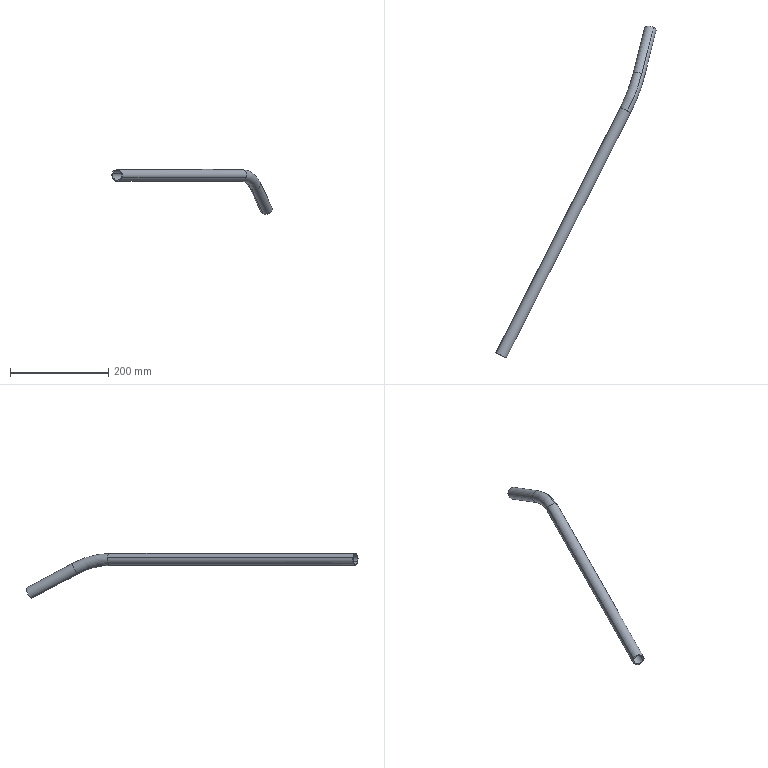Component | SolidWorks | ScribingMechanismAssembly-1_ScribingPlateMovableTube-1 | 1 solid | 14 faces | box 326.24 x 675.84 x 91.68 mm | volume 103418 mm3 | cylinder 8 | torus 4 | plane 2 | commonest cylinder face diameters 24 x4 20 x4
STEP:
#1=COLOUR_RGB('',0.7922,0.8196,0.9333);
#2=FILL_AREA_STYLE_COLOUR('',#1);
#3=FILL_AREA_STYLE('',(#2));
#4=SURFACE_STYLE_FILL_AREA(#3);
#5=SURFACE_SIDE_STYLE('',(#4));
#6=SURFACE_STYLE_USAGE(.BOTH.,#5);
#7=PRESENTATION_STYLE_ASSIGNMENT((#6));
#8=CARTESIAN_POINT('',(-5.227,-4.938,37.723));
#9=VERTEX_POINT('',#8);
#10=CARTESIAN_POINT('',(-5.042,-5.032,37.207));
#11=VERTEX_POINT('',#10);
#12=CARTESIAN_POINT('',(-5.365,-4.868,37.361));
#13=DIRECTION('',(0.4521,0.892,0.));
#14=DIRECTION('',(-0.8209,0.4161,0.3911));
#15=AXIS2_PLACEMENT_3D('',#12,#13,#14);
#16=CIRCLE('',#15,0.3937);
#17=EDGE_CURVE('',#9,#11,#16,.T.);
#18=ORIENTED_EDGE('',*,*,#17,.F.);
#19=CARTESIAN_POINT('',(-4.098,-1.979,36.947));
#20=VERTEX_POINT('',#19);
#21=CARTESIAN_POINT('',(-7.425,-3.824,31.926));
#22=DIRECTION('',(-0.8209,0.4161,0.3911));
#23=DIRECTION('',(-0.4521,-0.892,0.));
#24=AXIS2_PLACEMENT_3D('',#21,#22,#23);
#25=CIRCLE('',#24,6.299);
#26=EDGE_CURVE('',#9,#20,#25,.T.);
#27=ORIENTED_EDGE('',*,*,#26,.T.);
#28=CARTESIAN_POINT('',(-4.514,-2.21,36.319));
#29=VERTEX_POINT('',#28);
#30=CARTESIAN_POINT('',(-4.306,-2.095,36.633));
#31=DIRECTION('',(0.2171,0.8609,-0.4602));
#32=DIRECTION('',(-0.8209,0.4161,0.3911));
#33=AXIS2_PLACEMENT_3D('',#30,#31,#32);
#34=CIRCLE('',#33,0.3937);
#35=EDGE_CURVE('',#20,#29,#34,.T.);
#36=ORIENTED_EDGE('',*,*,#35,.T.);
#37=CARTESIAN_POINT('',(-5.502,-4.799,36.999));
#38=VERTEX_POINT('',#37);
#39=CARTESIAN_POINT('',(-7.425,-3.824,31.926));
#40=DIRECTION('',(-0.8209,0.4161,0.3911));
#41=DIRECTION('',(-0.4521,-0.892,0.));
#42=AXIS2_PLACEMENT_3D('',#39,#40,#41);
#43=CIRCLE('',#42,5.512);
#44=EDGE_CURVE('',#38,#29,#43,.T.);
#45=ORIENTED_EDGE('',*,*,#44,.F.);
#46=CARTESIAN_POINT('',(-5.365,-4.868,37.361));
#47=DIRECTION('',(0.4521,0.892,0.));
#48=DIRECTION('',(-0.8209,0.4161,0.3911));
#49=AXIS2_PLACEMENT_3D('',#46,#47,#48);
#50=CIRCLE('',#49,0.3937);
#51=EDGE_CURVE('',#11,#38,#50,.T.);
#52=ORIENTED_EDGE('',*,*,#51,.F.);
#53=EDGE_LOOP('',(#18,#27,#36,#45,#52));
#54=FACE_OUTER_BOUND('',#53,.T.);
#55=CARTESIAN_POINT('',(-7.425,-3.824,31.926));
#56=DIRECTION('',(-0.8209,0.4161,0.3911));
#57=DIRECTION('',(0.3489,-0.1768,0.9203));
#58=AXIS2_PLACEMENT_3D('',#55,#56,#57);
#59=TOROIDAL_SURFACE('',#58,5.906,0.3937);
#60=ADVANCED_FACE('',(#54),#59,.F.);
#61=CARTESIAN_POINT('',(-5.753,-4.672,37.546));
#62=VERTEX_POINT('',#61);
#63=CARTESIAN_POINT('',(-5.2,-4.952,37.796));
#64=VERTEX_POINT('',#63);
#65=CARTESIAN_POINT('',(-5.365,-4.868,37.361));
#66=DIRECTION('',(0.4521,0.892,0.));
#67=DIRECTION('',(-0.8209,0.4161,0.3911));
#68=AXIS2_PLACEMENT_3D('',#65,#66,#67);
#69=CIRCLE('',#68,0.4724);
#70=EDGE_CURVE('',#62,#64,#69,.T.);
#71=ORIENTED_EDGE('',*,*,#70,.T.);
#72=CARTESIAN_POINT('',(-4.056,-1.956,37.009));
#73=VERTEX_POINT('',#72);
#74=CARTESIAN_POINT('',(-7.425,-3.824,31.926));
#75=DIRECTION('',(-0.8209,0.4161,0.3911));
#76=DIRECTION('',(-0.4521,-0.892,0.));
#77=AXIS2_PLACEMENT_3D('',#74,#75,#76);
#78=CIRCLE('',#77,6.378);
#79=EDGE_CURVE('',#64,#73,#78,.T.);
#80=ORIENTED_EDGE('',*,*,#79,.T.);
#81=CARTESIAN_POINT('',(-4.555,-2.233,36.256));
#82=VERTEX_POINT('',#81);
#83=CARTESIAN_POINT('',(-4.306,-2.095,36.633));
#84=DIRECTION('',(0.2171,0.8609,-0.4602));
#85=DIRECTION('',(-0.8209,0.4161,0.3911));
#86=AXIS2_PLACEMENT_3D('',#83,#84,#85);
#87=CIRCLE('',#86,0.4724);
#88=EDGE_CURVE('',#82,#73,#87,.T.);
#89=ORIENTED_EDGE('',*,*,#88,.F.);
#90=CARTESIAN_POINT('',(-5.53,-4.785,36.926));
#91=VERTEX_POINT('',#90);
#92=CARTESIAN_POINT('',(-7.425,-3.824,31.926));
#93=DIRECTION('',(-0.8209,0.4161,0.3911));
#94=DIRECTION('',(-0.4521,-0.892,0.));
#95=AXIS2_PLACEMENT_3D('',#92,#93,#94);
#96=CIRCLE('',#95,5.433);
#97=EDGE_CURVE('',#91,#82,#96,.T.);
#98=ORIENTED_EDGE('',*,*,#97,.F.);
#99=CARTESIAN_POINT('',(-5.365,-4.868,37.361));
#100=DIRECTION('',(0.4521,0.892,0.));
#101=DIRECTION('',(-0.8209,0.4161,0.3911));
#102=AXIS2_PLACEMENT_3D('',#99,#100,#101);
#103=CIRCLE('',#102,0.4724);
#104=EDGE_CURVE('',#91,#62,#103,.T.);
#105=ORIENTED_EDGE('',*,*,#104,.T.);
#106=EDGE_LOOP('',(#71,#80,#89,#98,#105));
#107=FACE_OUTER_BOUND('',#106,.T.);
#108=CARTESIAN_POINT('',(-7.425,-3.824,31.926));
#109=DIRECTION('',(-0.8209,0.4161,0.3911));
#110=DIRECTION('',(0.3489,-0.1768,0.9203));
#111=AXIS2_PLACEMENT_3D('',#108,#109,#110);
#112=TOROIDAL_SURFACE('',#111,5.906,0.4724);
#113=ADVANCED_FACE('',(#107),#112,.T.);
#114=ORIENTED_EDGE('',*,*,#70,.F.);
#115=CARTESIAN_POINT('',(-15.717,-24.33,37.546));
#116=VERTEX_POINT('',#115);
#117=CARTESIAN_POINT('',(-5.753,-4.672,37.546));
#118=DIRECTION('',(-0.4521,-0.892,-0.));
#119=VECTOR('',#118,39.37);
#120=LINE('',#117,#119);
#121=EDGE_CURVE('',#62,#116,#120,.T.);
#122=ORIENTED_EDGE('',*,*,#121,.T.);
#123=CARTESIAN_POINT('',(-14.941,-24.724,37.176));
#124=VERTEX_POINT('',#123);
#125=CARTESIAN_POINT('',(-15.329,-24.527,37.361));
#126=DIRECTION('',(0.4521,0.892,0.));
#127=DIRECTION('',(-0.8209,0.4161,0.3911));
#128=AXIS2_PLACEMENT_3D('',#125,#126,#127);
#129=CIRCLE('',#128,0.4724);
#130=EDGE_CURVE('',#116,#124,#129,.T.);
#131=ORIENTED_EDGE('',*,*,#130,.T.);
#132=CARTESIAN_POINT('',(-4.977,-5.065,37.176));
#133=VERTEX_POINT('',#132);
#134=CARTESIAN_POINT('',(-4.977,-5.065,37.176));
#135=DIRECTION('',(-0.4521,-0.892,-0.));
#136=VECTOR('',#135,39.37);
#137=LINE('',#134,#136);
#138=EDGE_CURVE('',#133,#124,#137,.T.);
#139=ORIENTED_EDGE('',*,*,#138,.F.);
#140=CARTESIAN_POINT('',(-5.365,-4.868,37.361));
#141=DIRECTION('',(0.4521,0.892,0.));
#142=DIRECTION('',(-0.8209,0.4161,0.3911));
#143=AXIS2_PLACEMENT_3D('',#140,#141,#142);
#144=CIRCLE('',#143,0.4724);
#145=EDGE_CURVE('',#64,#133,#144,.T.);
#146=ORIENTED_EDGE('',*,*,#145,.F.);
#147=EDGE_LOOP('',(#114,#122,#131,#139,#146));
#148=FACE_OUTER_BOUND('',#147,.T.);
#149=CARTESIAN_POINT('',(-5.365,-4.868,37.361));
#150=DIRECTION('',(-0.4521,-0.892,-0.));
#151=DIRECTION('',(0.8209,-0.4161,-0.3911));
#152=AXIS2_PLACEMENT_3D('',#149,#150,#151);
#153=CYLINDRICAL_SURFACE('',#152,0.4724);
#154=ADVANCED_FACE('',(#148),#153,.T.);
#155=ORIENTED_EDGE('',*,*,#51,.T.);
#156=CARTESIAN_POINT('',(-5.688,-4.704,37.515));
#157=VERTEX_POINT('',#156);
#158=CARTESIAN_POINT('',(-5.365,-4.868,37.361));
#159=DIRECTION('',(0.4521,0.892,0.));
#160=DIRECTION('',(-0.8209,0.4161,0.3911));
#161=AXIS2_PLACEMENT_3D('',#158,#159,#160);
#162=CIRCLE('',#161,0.3937);
#163=EDGE_CURVE('',#38,#157,#162,.T.);
#164=ORIENTED_EDGE('',*,*,#163,.T.);
#165=CARTESIAN_POINT('',(-15.652,-24.363,37.515));
#166=VERTEX_POINT('',#165);
#167=CARTESIAN_POINT('',(-5.688,-4.704,37.515));
#168=DIRECTION('',(-0.4521,-0.892,-0.));
#169=VECTOR('',#168,39.37);
#170=LINE('',#167,#169);
#171=EDGE_CURVE('',#157,#166,#170,.T.);
#172=ORIENTED_EDGE('',*,*,#171,.T.);
#173=CARTESIAN_POINT('',(-15.006,-24.691,37.207));
#174=VERTEX_POINT('',#173);
#175=CARTESIAN_POINT('',(-15.329,-24.527,37.361));
#176=DIRECTION('',(0.4521,0.892,0.));
#177=DIRECTION('',(-0.8209,0.4161,0.3911));
#178=AXIS2_PLACEMENT_3D('',#175,#176,#177);
#179=CIRCLE('',#178,0.3937);
#180=EDGE_CURVE('',#174,#166,#179,.T.);
#181=ORIENTED_EDGE('',*,*,#180,.F.);
#182=CARTESIAN_POINT('',(-5.042,-5.032,37.207));
#183=DIRECTION('',(-0.4521,-0.892,-0.));
#184=VECTOR('',#183,39.37);
#185=LINE('',#182,#184);
#186=EDGE_CURVE('',#11,#174,#185,.T.);
#187=ORIENTED_EDGE('',*,*,#186,.F.);
#188=EDGE_LOOP('',(#155,#164,#172,#181,#187));
#189=FACE_OUTER_BOUND('',#188,.T.);
#190=CARTESIAN_POINT('',(-5.365,-4.868,37.361));
#191=DIRECTION('',(-0.4521,-0.892,-0.));
#192=DIRECTION('',(0.8209,-0.4161,-0.3911));
#193=AXIS2_PLACEMENT_3D('',#190,#191,#192);
#194=CYLINDRICAL_SURFACE('',#193,0.3937);
#195=ADVANCED_FACE('',(#189),#194,.F.);
#196=ORIENTED_EDGE('',*,*,#35,.F.);
#197=CARTESIAN_POINT('',(-3.159,1.742,34.957));
#198=VERTEX_POINT('',#197);
#199=CARTESIAN_POINT('',(-4.098,-1.979,36.947));
#200=DIRECTION('',(0.2171,0.8609,-0.4602));
#201=VECTOR('',#200,39.37);
#202=LINE('',#199,#201);
#203=EDGE_CURVE('',#20,#198,#202,.T.);
#204=ORIENTED_EDGE('',*,*,#203,.T.);
#205=CARTESIAN_POINT('',(-3.575,1.512,34.33));
#206=VERTEX_POINT('',#205);
#207=CARTESIAN_POINT('',(-3.367,1.627,34.644));
#208=DIRECTION('',(0.2171,0.8609,-0.4602));
#209=DIRECTION('',(-0.8209,0.4161,0.3911));
#210=AXIS2_PLACEMENT_3D('',#207,#208,#209);
#211=CIRCLE('',#210,0.3937);
#212=EDGE_CURVE('',#198,#206,#211,.T.);
#213=ORIENTED_EDGE('',*,*,#212,.T.);
#214=CARTESIAN_POINT('',(-4.514,-2.21,36.319));
#215=DIRECTION('',(0.2171,0.8609,-0.4602));
#216=VECTOR('',#215,39.37);
#217=LINE('',#214,#216);
#218=EDGE_CURVE('',#29,#206,#217,.T.);
#219=ORIENTED_EDGE('',*,*,#218,.F.);
#220=EDGE_LOOP('',(#196,#204,#213,#219));
#221=FACE_OUTER_BOUND('',#220,.T.);
#222=CARTESIAN_POINT('',(-4.306,-2.095,36.633));
#223=DIRECTION('',(0.2171,0.8609,-0.4602));
#224=DIRECTION('',(-0.5282,-0.2928,-0.797));
#225=AXIS2_PLACEMENT_3D('',#222,#223,#224);
#226=CYLINDRICAL_SURFACE('',#225,0.3937);
#227=ADVANCED_FACE('',(#221),#226,.F.);
#228=ORIENTED_EDGE('',*,*,#88,.T.);
#229=CARTESIAN_POINT('',(-3.118,1.765,35.02));
#230=VERTEX_POINT('',#229);
#231=CARTESIAN_POINT('',(-4.056,-1.956,37.009));
#232=DIRECTION('',(0.2171,0.8609,-0.4602));
#233=VECTOR('',#232,39.37);
#234=LINE('',#231,#233);
#235=EDGE_CURVE('',#73,#230,#234,.T.);
#236=ORIENTED_EDGE('',*,*,#235,.T.);
#237=CARTESIAN_POINT('',(-3.617,1.489,34.267));
#238=VERTEX_POINT('',#237);
#239=CARTESIAN_POINT('',(-3.367,1.627,34.644));
#240=DIRECTION('',(0.2171,0.8609,-0.4602));
#241=DIRECTION('',(-0.8209,0.4161,0.3911));
#242=AXIS2_PLACEMENT_3D('',#239,#240,#241);
#243=CIRCLE('',#242,0.4724);
#244=EDGE_CURVE('',#238,#230,#243,.T.);
#245=ORIENTED_EDGE('',*,*,#244,.F.);
#246=CARTESIAN_POINT('',(-4.555,-2.233,36.256));
#247=DIRECTION('',(0.2171,0.8609,-0.4602));
#248=VECTOR('',#247,39.37);
#249=LINE('',#246,#248);
#250=EDGE_CURVE('',#82,#238,#249,.T.);
#251=ORIENTED_EDGE('',*,*,#250,.F.);
#252=EDGE_LOOP('',(#228,#236,#245,#251));
#253=FACE_OUTER_BOUND('',#252,.T.);
#254=CARTESIAN_POINT('',(-4.306,-2.095,36.633));
#255=DIRECTION('',(0.2171,0.8609,-0.4602));
#256=DIRECTION('',(-0.5282,-0.2928,-0.797));
#257=AXIS2_PLACEMENT_3D('',#254,#255,#256);
#258=CYLINDRICAL_SURFACE('',#257,0.4724);
#259=ADVANCED_FACE('',(#253),#258,.T.);
#260=ORIENTED_EDGE('',*,*,#235,.F.);
#261=CARTESIAN_POINT('',(-4.306,-2.095,36.633));
#262=DIRECTION('',(0.2171,0.8609,-0.4602));
#263=DIRECTION('',(-0.8209,0.4161,0.3911));
#264=AXIS2_PLACEMENT_3D('',#261,#262,#263);
#265=CIRCLE('',#264,0.4724);
#266=EDGE_CURVE('',#73,#82,#265,.T.);
#267=ORIENTED_EDGE('',*,*,#266,.T.);
#268=ORIENTED_EDGE('',*,*,#250,.T.);
#269=CARTESIAN_POINT('',(-3.367,1.627,34.644));
#270=DIRECTION('',(0.2171,0.8609,-0.4602));
#271=DIRECTION('',(-0.8209,0.4161,0.3911));
#272=AXIS2_PLACEMENT_3D('',#269,#270,#271);
#273=CIRCLE('',#272,0.4724);
#274=EDGE_CURVE('',#230,#238,#273,.T.);
#275=ORIENTED_EDGE('',*,*,#274,.F.);
#276=EDGE_LOOP('',(#260,#267,#268,#275));
#277=FACE_OUTER_BOUND('',#276,.T.);
#278=CARTESIAN_POINT('',(-4.306,-2.095,36.633));
#279=DIRECTION('',(0.2171,0.8609,-0.4602));
#280=DIRECTION('',(-0.5282,-0.2928,-0.797));
#281=AXIS2_PLACEMENT_3D('',#278,#279,#280);
#282=CYLINDRICAL_SURFACE('',#281,0.4724);
#283=ADVANCED_FACE('',(#277),#282,.T.);
#284=ORIENTED_EDGE('',*,*,#203,.F.);
#285=CARTESIAN_POINT('',(-4.306,-2.095,36.633));
#286=DIRECTION('',(0.2171,0.8609,-0.4602));
#287=DIRECTION('',(-0.8209,0.4161,0.3911));
#288=AXIS2_PLACEMENT_3D('',#285,#286,#287);
#289=CIRCLE('',#288,0.3937);
#290=EDGE_CURVE('',#29,#20,#289,.T.);
#291=ORIENTED_EDGE('',*,*,#290,.F.);
#292=ORIENTED_EDGE('',*,*,#218,.T.);
#293=CARTESIAN_POINT('',(-3.367,1.627,34.644));
#294=DIRECTION('',(0.2171,0.8609,-0.4602));
#295=DIRECTION('',(-0.8209,0.4161,0.3911));
#296=AXIS2_PLACEMENT_3D('',#293,#294,#295);
#297=CIRCLE('',#296,0.3937);
#298=EDGE_CURVE('',#206,#198,#297,.T.);
#299=ORIENTED_EDGE('',*,*,#298,.T.);
#300=EDGE_LOOP('',(#284,#291,#292,#299));
#301=FACE_OUTER_BOUND('',#300,.T.);
#302=CARTESIAN_POINT('',(-4.306,-2.095,36.633));
#303=DIRECTION('',(0.2171,0.8609,-0.4602));
#304=DIRECTION('',(-0.5282,-0.2928,-0.797));
#305=AXIS2_PLACEMENT_3D('',#302,#303,#304);
#306=CYLINDRICAL_SURFACE('',#305,0.3937);
#307=ADVANCED_FACE('',(#301),#306,.F.);
#308=ORIENTED_EDGE('',*,*,#79,.F.);
#309=ORIENTED_EDGE('',*,*,#145,.T.);
#310=CARTESIAN_POINT('',(-5.365,-4.868,37.361));
#311=DIRECTION('',(0.4521,0.892,0.));
#312=DIRECTION('',(-0.8209,0.4161,0.3911));
#313=AXIS2_PLACEMENT_3D('',#310,#311,#312);
#314=CIRCLE('',#313,0.4724);
#315=EDGE_CURVE('',#133,#91,#314,.T.);
#316=ORIENTED_EDGE('',*,*,#315,.T.);
#317=ORIENTED_EDGE('',*,*,#97,.T.);
#318=ORIENTED_EDGE('',*,*,#266,.F.);
#319=EDGE_LOOP('',(#308,#309,#316,#317,#318));
#320=FACE_OUTER_BOUND('',#319,.T.);
#321=CARTESIAN_POINT('',(-7.425,-3.824,31.926));
#322=DIRECTION('',(-0.8209,0.4161,0.3911));
#323=DIRECTION('',(0.3489,-0.1768,0.9203));
#324=AXIS2_PLACEMENT_3D('',#321,#322,#323);
#325=TOROIDAL_SURFACE('',#324,5.906,0.4724);
#326=ADVANCED_FACE('',(#320),#325,.T.);
#327=ORIENTED_EDGE('',*,*,#26,.F.);
#328=CARTESIAN_POINT('',(-5.365,-4.868,37.361));
#329=DIRECTION('',(0.4521,0.892,0.));
#330=DIRECTION('',(-0.8209,0.4161,0.3911));
#331=AXIS2_PLACEMENT_3D('',#328,#329,#330);
#332=CIRCLE('',#331,0.3937);
#333=EDGE_CURVE('',#157,#9,#332,.T.);
#334=ORIENTED_EDGE('',*,*,#333,.F.);
#335=ORIENTED_EDGE('',*,*,#163,.F.);
#336=ORIENTED_EDGE('',*,*,#44,.T.);
#337=ORIENTED_EDGE('',*,*,#290,.T.);
#338=EDGE_LOOP('',(#327,#334,#335,#336,#337));
#339=FACE_OUTER_BOUND('',#338,.T.);
#340=CARTESIAN_POINT('',(-7.425,-3.824,31.926));
#341=DIRECTION('',(-0.8209,0.4161,0.3911));
#342=DIRECTION('',(0.3489,-0.1768,0.9203));
#343=AXIS2_PLACEMENT_3D('',#340,#341,#342);
#344=TOROIDAL_SURFACE('',#343,5.906,0.3937);
#345=ADVANCED_FACE('',(#339),#344,.F.);
#346=ORIENTED_EDGE('',*,*,#171,.F.);
#347=ORIENTED_EDGE('',*,*,#333,.T.);
#348=ORIENTED_EDGE('',*,*,#17,.T.);
#349=ORIENTED_EDGE('',*,*,#186,.T.);
#350=CARTESIAN_POINT('',(-15.329,-24.527,37.361));
#351=DIRECTION('',(0.4521,0.892,0.));
#352=DIRECTION('',(-0.8209,0.4161,0.3911));
#353=AXIS2_PLACEMENT_3D('',#350,#351,#352);
#354=CIRCLE('',#353,0.3937);
#355=EDGE_CURVE('',#166,#174,#354,.T.);
#356=ORIENTED_EDGE('',*,*,#355,.F.);
#357=EDGE_LOOP('',(#346,#347,#348,#349,#356));
#358=FACE_OUTER_BOUND('',#357,.T.);
#359=CARTESIAN_POINT('',(-5.365,-4.868,37.361));
#360=DIRECTION('',(-0.4521,-0.892,-0.));
#361=DIRECTION('',(0.8209,-0.4161,-0.3911));
#362=AXIS2_PLACEMENT_3D('',#359,#360,#361);
#363=CYLINDRICAL_SURFACE('',#362,0.3937);
#364=ADVANCED_FACE('',(#358),#363,.F.);
#365=ORIENTED_EDGE('',*,*,#121,.F.);
#366=ORIENTED_EDGE('',*,*,#104,.F.);
#367=ORIENTED_EDGE('',*,*,#315,.F.);
#368=ORIENTED_EDGE('',*,*,#138,.T.);
#369=CARTESIAN_POINT('',(-15.329,-24.527,37.361));
#370=DIRECTION('',(0.4521,0.892,0.));
#371=DIRECTION('',(-0.8209,0.4161,0.3911));
#372=AXIS2_PLACEMENT_3D('',#369,#370,#371);
#373=CIRCLE('',#372,0.4724);
#374=EDGE_CURVE('',#124,#116,#373,.T.);
#375=ORIENTED_EDGE('',*,*,#374,.T.);
#376=EDGE_LOOP('',(#365,#366,#367,#368,#375));
#377=FACE_OUTER_BOUND('',#376,.T.);
#378=CARTESIAN_POINT('',(-5.365,-4.868,37.361));
#379=DIRECTION('',(-0.4521,-0.892,-0.));
#380=DIRECTION('',(0.8209,-0.4161,-0.3911));
#381=AXIS2_PLACEMENT_3D('',#378,#379,#380);
#382=CYLINDRICAL_SURFACE('',#381,0.4724);
#383=ADVANCED_FACE('',(#377),#382,.T.);
#384=ORIENTED_EDGE('',*,*,#298,.F.);
#385=ORIENTED_EDGE('',*,*,#212,.F.);
#386=EDGE_LOOP('',(#384,#385));
#387=FACE_BOUND('',#386,.T.);
#388=ORIENTED_EDGE('',*,*,#244,.T.);
#389=ORIENTED_EDGE('',*,*,#274,.T.);
#390=EDGE_LOOP('',(#388,#389));
#391=FACE_OUTER_BOUND('',#390,.T.);
#392=CARTESIAN_POINT('',(-3.367,1.627,34.644));
#393=DIRECTION('',(0.2171,0.8609,-0.4602));
#394=DIRECTION('',(-0.8209,0.4161,0.3911));
#395=AXIS2_PLACEMENT_3D('',#392,#393,#394);
#396=PLANE('',#395);
#397=ADVANCED_FACE('',(#387,#391),#396,.T.);
#398=ORIENTED_EDGE('',*,*,#180,.T.);
#399=ORIENTED_EDGE('',*,*,#355,.T.);
#400=EDGE_LOOP('',(#398,#399));
#401=FACE_BOUND('',#400,.T.);
#402=ORIENTED_EDGE('',*,*,#374,.F.);
#403=ORIENTED_EDGE('',*,*,#130,.F.);
#404=EDGE_LOOP('',(#402,#403));
#405=FACE_OUTER_BOUND('',#404,.T.);
#406=CARTESIAN_POINT('',(-15.329,-24.527,37.361));
#407=DIRECTION('',(0.4521,0.892,0.));
#408=DIRECTION('',(-0.8209,0.4161,0.3911));
#409=AXIS2_PLACEMENT_3D('',#406,#407,#408);
#410=PLANE('',#409);
#411=ADVANCED_FACE('',(#401,#405),#410,.F.);
#412=CLOSED_SHELL('',(#60,#113,#154,#195,#227,#259,#283,#307,#326,#345,#364,#383,#397,#411));
#413=MANIFOLD_SOLID_BREP('',#412);
#414=STYLED_ITEM('',(#7),#413);
#415=PRESENTATION_LAYER_ASSIGNMENT('','',(#414));
#416=CARTESIAN_POINT('',(0.,0.,0.));
#417=DIRECTION('',(0.,0.,1.));
#418=DIRECTION('',(1.,0.,0.));
#419=AXIS2_PLACEMENT_3D('',#416,#417,#418);
#420=(LENGTH_UNIT()NAMED_UNIT(*)SI_UNIT($,.METRE.));
#421=LENGTH_MEASURE_WITH_UNIT(LENGTH_MEASURE(0.0254),#420);
#422=DIMENSIONAL_EXPONENTS(1.,0.,0.,0.,0.,0.,0.);
#423=(CONVERSION_BASED_UNIT('',#421)LENGTH_UNIT()NAMED_UNIT(#422));
#424=UNCERTAINTY_MEASURE_WITH_UNIT(LENGTH_MEASURE(0.00001),#423,'','');
#425=(NAMED_UNIT(*)PLANE_ANGLE_UNIT()SI_UNIT($,.RADIAN.));
#426=(NAMED_UNIT(*)SI_UNIT($,.STERADIAN.)SOLID_ANGLE_UNIT());
#427=(GEOMETRIC_REPRESENTATION_CONTEXT(3)GLOBAL_UNCERTAINTY_ASSIGNED_CONTEXT((#424))GLOBAL_UNIT_ASSIGNED_CONTEXT((#423,#425,#426))REPRESENTATION_CONTEXT('',''));
#428=ADVANCED_BREP_SHAPE_REPRESENTATION('',(#413,#419),#427);
#429=(LENGTH_UNIT()NAMED_UNIT(*)SI_UNIT($,.METRE.));
#430=LENGTH_MEASURE_WITH_UNIT(LENGTH_MEASURE(0.0254),#429);
#431=DIMENSIONAL_EXPONENTS(1.,0.,0.,0.,0.,0.,0.);
#432=(CONVERSION_BASED_UNIT('',#430)LENGTH_UNIT()NAMED_UNIT(#431));
#433=UNCERTAINTY_MEASURE_WITH_UNIT(LENGTH_MEASURE(0.00001),#432,'','');
#434=(NAMED_UNIT(*)PLANE_ANGLE_UNIT()SI_UNIT($,.RADIAN.));
#435=(NAMED_UNIT(*)SI_UNIT($,.STERADIAN.)SOLID_ANGLE_UNIT());
#436=(GEOMETRIC_REPRESENTATION_CONTEXT(3)GLOBAL_UNCERTAINTY_ASSIGNED_CONTEXT((#433))GLOBAL_UNIT_ASSIGNED_CONTEXT((#432,#434,#435))REPRESENTATION_CONTEXT('',''));
#437=MECHANICAL_DESIGN_GEOMETRIC_PRESENTATION_REPRESENTATION('',(#414),#436);